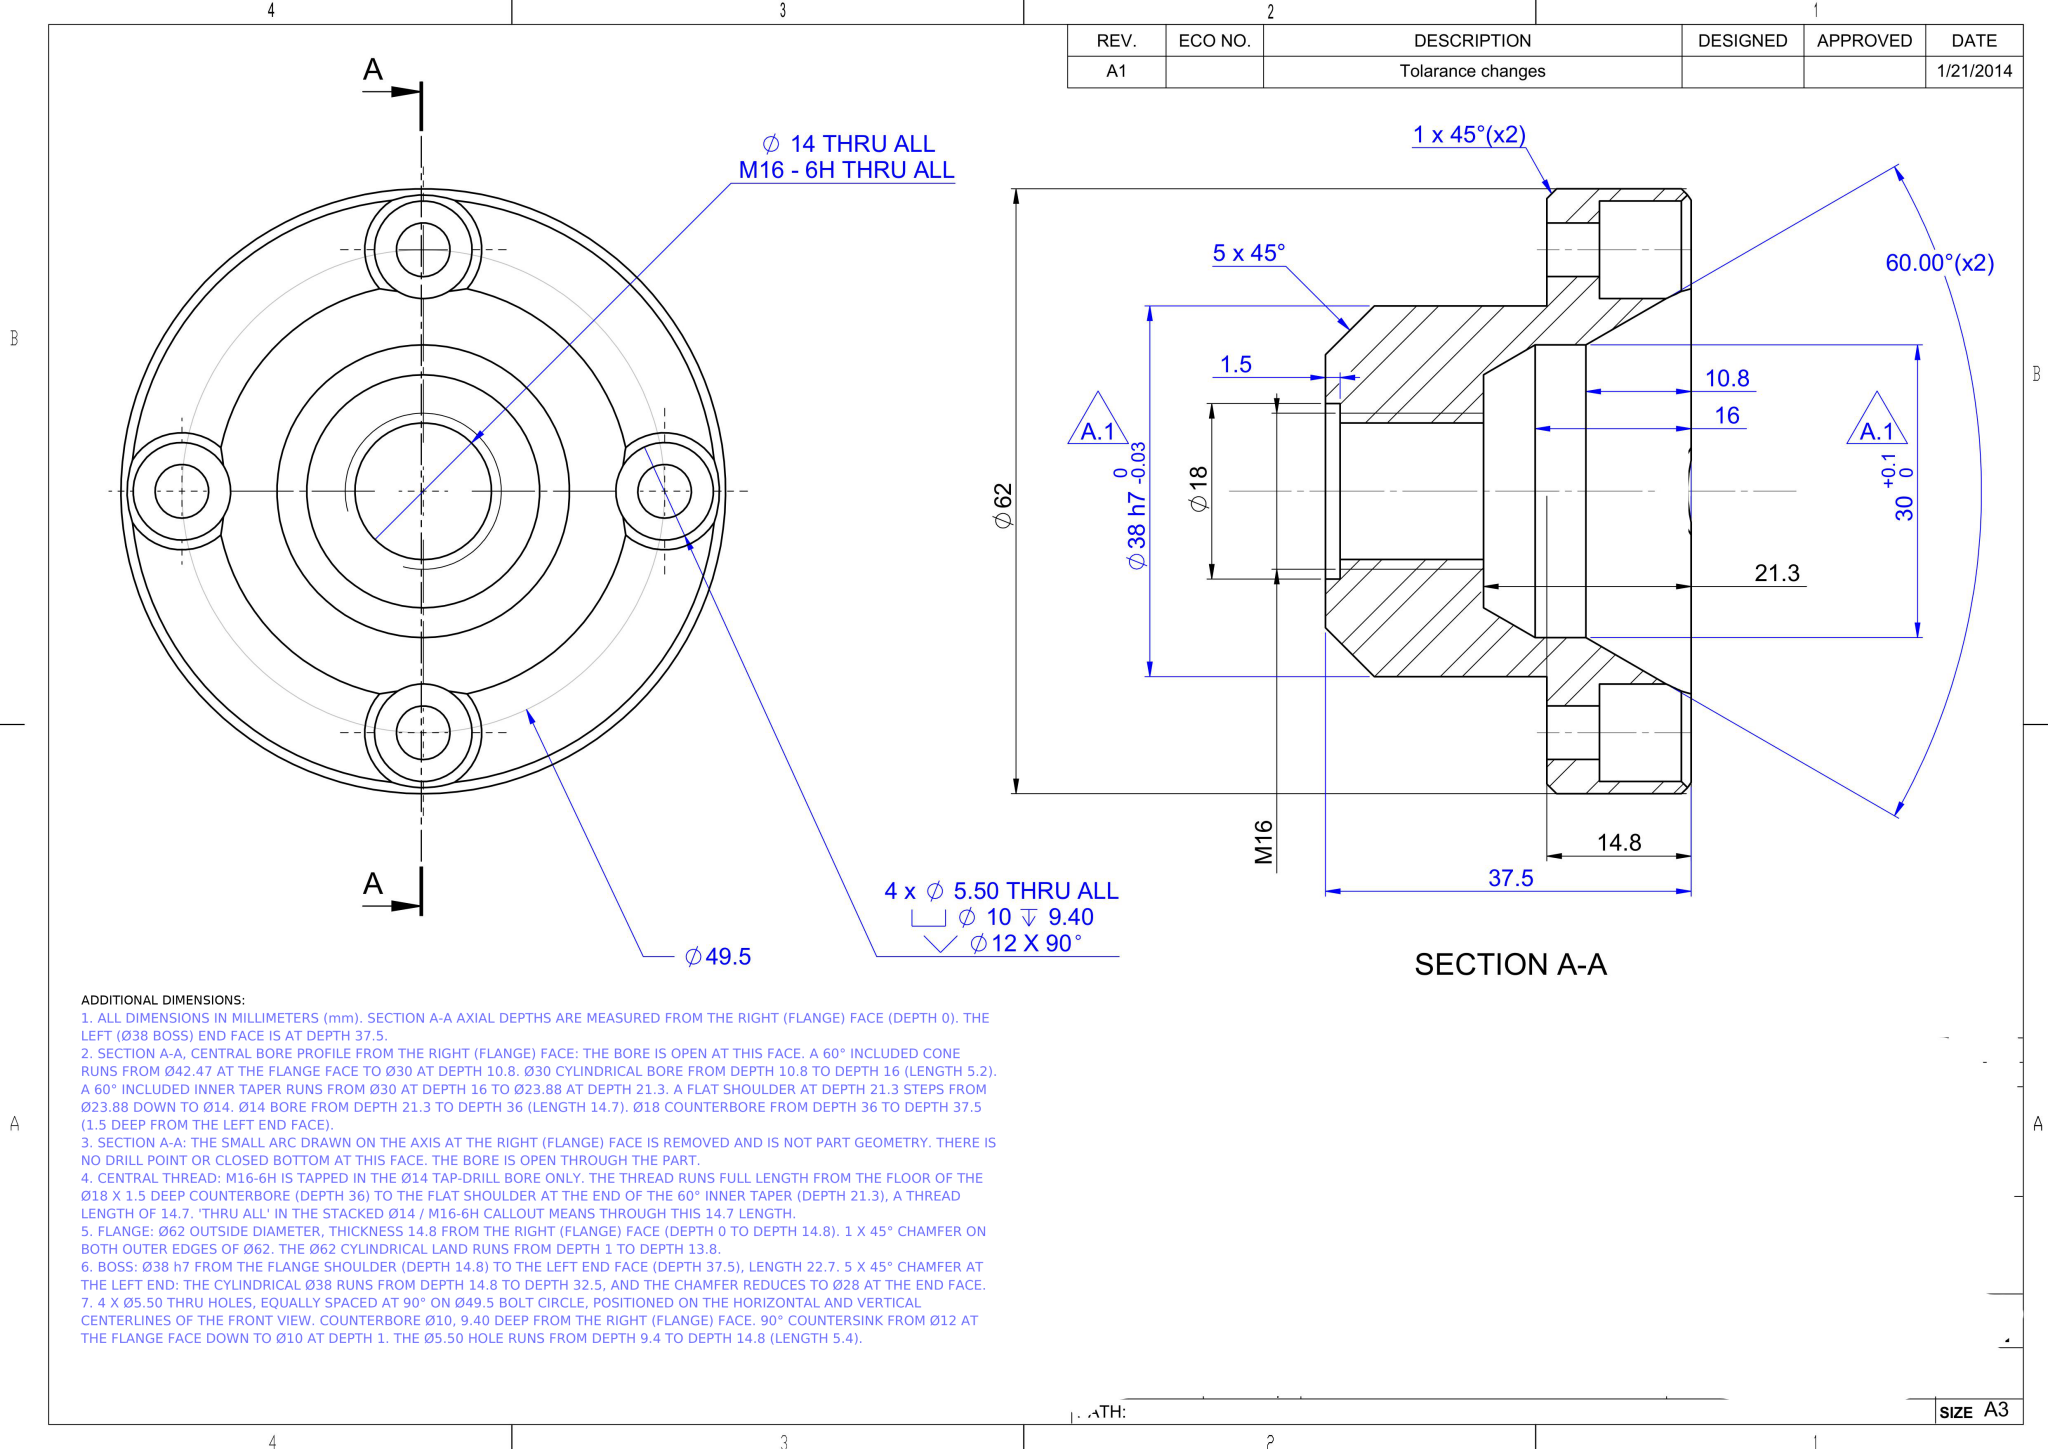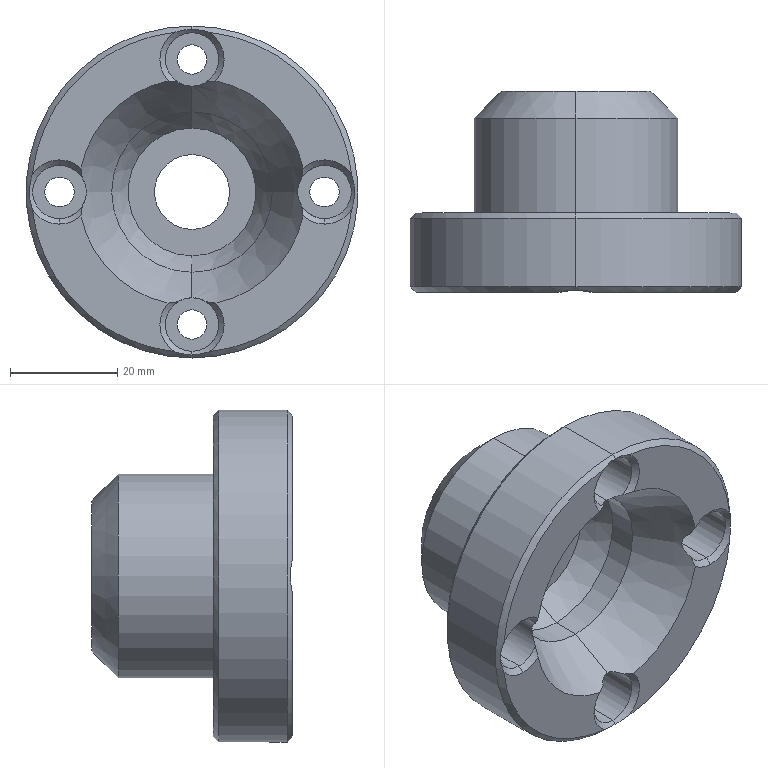Part | NX | mm | 1 solid | 57 faces | box 62 x 37.5 x 62 mm | volume 44783 mm3 | cylinder 26 | cone 19 | plane 12 | commonest cylinder face diameters 10 x8 5.5 x8 18 x2 30 x2 62 x2 38 x2 14 x2